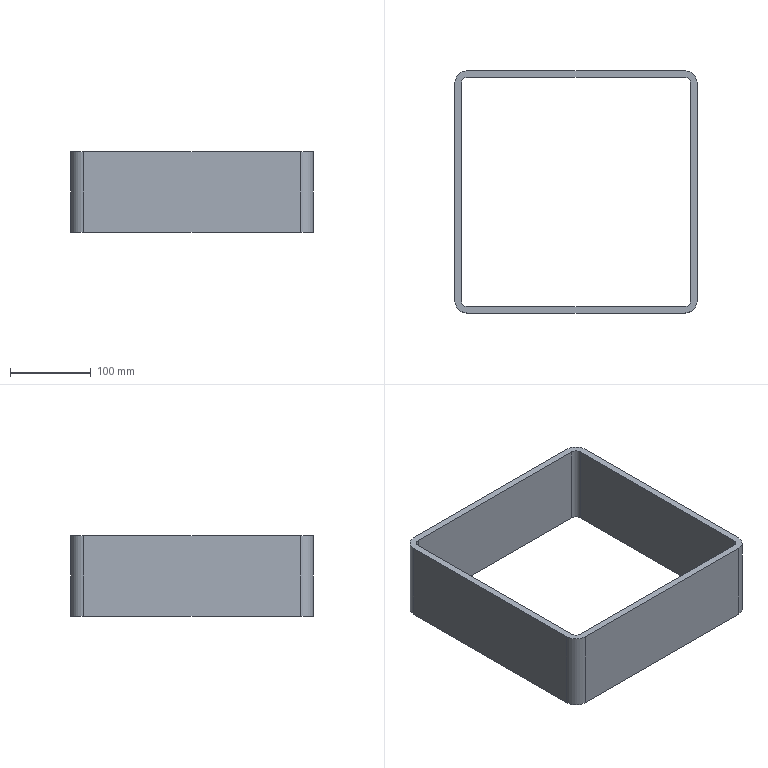Component | SolidWorks | TrolleyLeg-1_300 x 300 x 8-100-2 | 1 solid | 18 faces | box 300 x 300 x 100 mm | volume 917919 mm3 | plane 10 | cylinder 8 | commonest cylinder face diameters 32 x4 16 x4 | material Plain Carbon Steel
build123d program:
from build123d import *

# Parameters (mm, degrees)
BOSS_EXTRUDE1_DEPTH = 100


with BuildPart() as part:
    # Sketch1 → Boss-Extrude1 (new body)
    with BuildSketch(Plane.XY):
        with BuildLine():
            Line((-134, -150), (134, -150))
            ThreePointArc((134, -150), (145.314, -145.314), (150, -134))
            Line((150, -134), (150, 134))
            ThreePointArc((150, 134), (145.314, 145.314), (134, 150))
            Line((134, 150), (-134, 150))
            ThreePointArc((-134, 150), (-145.314, 145.314), (-150, 134))
            Line((-150, 134), (-150, -134))
            ThreePointArc((-150, -134), (-145.314, -145.314), (-134, -150))
        make_face()
        with BuildLine():
            Line((-134, -142), (134, -142))
            ThreePointArc((134, -142), (139.657, -139.657), (142, -134))
            Line((142, -134), (142, 134))
            ThreePointArc((142, 134), (139.657, 139.657), (134, 142))
            Line((134, 142), (-134, 142))
            ThreePointArc((-134, 142), (-139.657, 139.657), (-142, 134))
            Line((-142, 134), (-142, -134))
            ThreePointArc((-142, -134), (-139.657, -139.657), (-134, -142))
        make_face(mode=Mode.SUBTRACT)
    extrude(amount=BOSS_EXTRUDE1_DEPTH)


solid = part.part

# Placed as in the assembly
solid = solid.moved(Location((-2662.199, 1921.323, 3105.973), (0, 0, 0)))
STEP:
#1=COLOUR_RGB('',0.7922,0.8196,0.9333);
#2=FILL_AREA_STYLE_COLOUR('',#1);
#3=FILL_AREA_STYLE('',(#2));
#4=SURFACE_STYLE_FILL_AREA(#3);
#5=SURFACE_SIDE_STYLE('',(#4));
#6=SURFACE_STYLE_USAGE(.BOTH.,#5);
#7=PRESENTATION_STYLE_ASSIGNMENT((#6));
#8=CARTESIAN_POINT('',(-110.717,80.918,122.282));
#9=VERTEX_POINT('',#8);
#10=CARTESIAN_POINT('',(-110.087,81.548,122.282));
#11=VERTEX_POINT('',#10);
#12=CARTESIAN_POINT('',(-110.087,80.918,122.282));
#13=DIRECTION('',(0.,0.,-1.));
#14=DIRECTION('',(1.,0.,0.));
#15=AXIS2_PLACEMENT_3D('',#12,#13,#14);
#16=CIRCLE('',#15,0.6299);
#17=EDGE_CURVE('',#9,#11,#16,.T.);
#18=ORIENTED_EDGE('',*,*,#17,.T.);
#19=CARTESIAN_POINT('',(-99.535,81.548,122.282));
#20=VERTEX_POINT('',#19);
#21=CARTESIAN_POINT('',(-110.087,81.548,122.282));
#22=DIRECTION('',(1.,0.,0.));
#23=VECTOR('',#22,39.37);
#24=LINE('',#21,#23);
#25=EDGE_CURVE('',#11,#20,#24,.T.);
#26=ORIENTED_EDGE('',*,*,#25,.T.);
#27=CARTESIAN_POINT('',(-98.905,80.918,122.282));
#28=VERTEX_POINT('',#27);
#29=CARTESIAN_POINT('',(-99.535,80.918,122.282));
#30=DIRECTION('',(0.,0.,-1.));
#31=DIRECTION('',(1.,0.,0.));
#32=AXIS2_PLACEMENT_3D('',#29,#30,#31);
#33=CIRCLE('',#32,0.6299);
#34=EDGE_CURVE('',#20,#28,#33,.T.);
#35=ORIENTED_EDGE('',*,*,#34,.T.);
#36=CARTESIAN_POINT('',(-98.905,70.367,122.282));
#37=VERTEX_POINT('',#36);
#38=CARTESIAN_POINT('',(-98.905,70.367,122.282));
#39=DIRECTION('',(0.,1.,0.));
#40=VECTOR('',#39,39.37);
#41=LINE('',#38,#40);
#42=EDGE_CURVE('',#37,#28,#41,.T.);
#43=ORIENTED_EDGE('',*,*,#42,.F.);
#44=CARTESIAN_POINT('',(-99.535,69.737,122.282));
#45=VERTEX_POINT('',#44);
#46=CARTESIAN_POINT('',(-99.535,70.367,122.282));
#47=DIRECTION('',(0.,0.,-1.));
#48=DIRECTION('',(1.,0.,0.));
#49=AXIS2_PLACEMENT_3D('',#46,#47,#48);
#50=CIRCLE('',#49,0.6299);
#51=EDGE_CURVE('',#37,#45,#50,.T.);
#52=ORIENTED_EDGE('',*,*,#51,.T.);
#53=CARTESIAN_POINT('',(-110.087,69.737,122.282));
#54=VERTEX_POINT('',#53);
#55=CARTESIAN_POINT('',(-99.535,69.737,122.282));
#56=DIRECTION('',(-1.,0.,0.));
#57=VECTOR('',#56,39.37);
#58=LINE('',#55,#57);
#59=EDGE_CURVE('',#45,#54,#58,.T.);
#60=ORIENTED_EDGE('',*,*,#59,.T.);
#61=CARTESIAN_POINT('',(-110.717,70.367,122.282));
#62=VERTEX_POINT('',#61);
#63=CARTESIAN_POINT('',(-110.087,70.367,122.282));
#64=DIRECTION('',(0.,0.,-1.));
#65=DIRECTION('',(1.,0.,0.));
#66=AXIS2_PLACEMENT_3D('',#63,#64,#65);
#67=CIRCLE('',#66,0.6299);
#68=EDGE_CURVE('',#54,#62,#67,.T.);
#69=ORIENTED_EDGE('',*,*,#68,.T.);
#70=CARTESIAN_POINT('',(-110.717,80.918,122.282));
#71=DIRECTION('',(0.,-1.,0.));
#72=VECTOR('',#71,39.37);
#73=LINE('',#70,#72);
#74=EDGE_CURVE('',#9,#62,#73,.T.);
#75=ORIENTED_EDGE('',*,*,#74,.F.);
#76=EDGE_LOOP('',(#18,#26,#35,#43,#52,#60,#69,#75));
#77=FACE_OUTER_BOUND('',#76,.T.);
#78=CARTESIAN_POINT('',(-110.087,81.233,122.282));
#79=VERTEX_POINT('',#78);
#80=CARTESIAN_POINT('',(-99.535,81.233,122.282));
#81=VERTEX_POINT('',#80);
#82=CARTESIAN_POINT('',(-110.087,81.233,122.282));
#83=DIRECTION('',(1.,0.,0.));
#84=VECTOR('',#83,39.37);
#85=LINE('',#82,#84);
#86=EDGE_CURVE('',#79,#81,#85,.T.);
#87=ORIENTED_EDGE('',*,*,#86,.F.);
#88=CARTESIAN_POINT('',(-110.402,80.918,122.282));
#89=VERTEX_POINT('',#88);
#90=CARTESIAN_POINT('',(-110.087,80.918,122.282));
#91=DIRECTION('',(0.,0.,-1.));
#92=DIRECTION('',(1.,0.,0.));
#93=AXIS2_PLACEMENT_3D('',#90,#91,#92);
#94=CIRCLE('',#93,0.315);
#95=EDGE_CURVE('',#89,#79,#94,.T.);
#96=ORIENTED_EDGE('',*,*,#95,.F.);
#97=CARTESIAN_POINT('',(-110.402,70.367,122.282));
#98=VERTEX_POINT('',#97);
#99=CARTESIAN_POINT('',(-110.402,80.918,122.282));
#100=DIRECTION('',(0.,-1.,0.));
#101=VECTOR('',#100,39.37);
#102=LINE('',#99,#101);
#103=EDGE_CURVE('',#89,#98,#102,.T.);
#104=ORIENTED_EDGE('',*,*,#103,.T.);
#105=CARTESIAN_POINT('',(-110.087,70.052,122.282));
#106=VERTEX_POINT('',#105);
#107=CARTESIAN_POINT('',(-110.087,70.367,122.282));
#108=DIRECTION('',(0.,0.,-1.));
#109=DIRECTION('',(1.,0.,0.));
#110=AXIS2_PLACEMENT_3D('',#107,#108,#109);
#111=CIRCLE('',#110,0.315);
#112=EDGE_CURVE('',#106,#98,#111,.T.);
#113=ORIENTED_EDGE('',*,*,#112,.F.);
#114=CARTESIAN_POINT('',(-99.535,70.052,122.282));
#115=VERTEX_POINT('',#114);
#116=CARTESIAN_POINT('',(-99.535,70.052,122.282));
#117=DIRECTION('',(-1.,0.,0.));
#118=VECTOR('',#117,39.37);
#119=LINE('',#116,#118);
#120=EDGE_CURVE('',#115,#106,#119,.T.);
#121=ORIENTED_EDGE('',*,*,#120,.F.);
#122=CARTESIAN_POINT('',(-99.22,70.367,122.282));
#123=VERTEX_POINT('',#122);
#124=CARTESIAN_POINT('',(-99.535,70.367,122.282));
#125=DIRECTION('',(0.,0.,-1.));
#126=DIRECTION('',(1.,0.,0.));
#127=AXIS2_PLACEMENT_3D('',#124,#125,#126);
#128=CIRCLE('',#127,0.315);
#129=EDGE_CURVE('',#123,#115,#128,.T.);
#130=ORIENTED_EDGE('',*,*,#129,.F.);
#131=CARTESIAN_POINT('',(-99.22,80.918,122.282));
#132=VERTEX_POINT('',#131);
#133=CARTESIAN_POINT('',(-99.22,70.367,122.282));
#134=DIRECTION('',(0.,1.,0.));
#135=VECTOR('',#134,39.37);
#136=LINE('',#133,#135);
#137=EDGE_CURVE('',#123,#132,#136,.T.);
#138=ORIENTED_EDGE('',*,*,#137,.T.);
#139=CARTESIAN_POINT('',(-99.535,80.918,122.282));
#140=DIRECTION('',(0.,0.,-1.));
#141=DIRECTION('',(1.,0.,0.));
#142=AXIS2_PLACEMENT_3D('',#139,#140,#141);
#143=CIRCLE('',#142,0.315);
#144=EDGE_CURVE('',#81,#132,#143,.T.);
#145=ORIENTED_EDGE('',*,*,#144,.F.);
#146=EDGE_LOOP('',(#87,#96,#104,#113,#121,#130,#138,#145));
#147=FACE_BOUND('',#146,.T.);
#148=CARTESIAN_POINT('',(-110.087,80.918,122.282));
#149=DIRECTION('',(0.,0.,-1.));
#150=DIRECTION('',(1.,0.,0.));
#151=AXIS2_PLACEMENT_3D('',#148,#149,#150);
#152=PLANE('',#151);
#153=ADVANCED_FACE('',(#77,#147),#152,.T.);
#154=CARTESIAN_POINT('',(-110.717,80.918,126.219));
#155=VERTEX_POINT('',#154);
#156=CARTESIAN_POINT('',(-110.087,81.548,126.219));
#157=VERTEX_POINT('',#156);
#158=CARTESIAN_POINT('',(-110.087,80.918,126.219));
#159=DIRECTION('',(0.,0.,-1.));
#160=DIRECTION('',(1.,0.,0.));
#161=AXIS2_PLACEMENT_3D('',#158,#159,#160);
#162=CIRCLE('',#161,0.6299);
#163=EDGE_CURVE('',#155,#157,#162,.T.);
#164=ORIENTED_EDGE('',*,*,#163,.F.);
#165=CARTESIAN_POINT('',(-110.717,70.367,126.219));
#166=VERTEX_POINT('',#165);
#167=CARTESIAN_POINT('',(-110.717,80.918,126.219));
#168=DIRECTION('',(0.,-1.,0.));
#169=VECTOR('',#168,39.37);
#170=LINE('',#167,#169);
#171=EDGE_CURVE('',#155,#166,#170,.T.);
#172=ORIENTED_EDGE('',*,*,#171,.T.);
#173=CARTESIAN_POINT('',(-110.087,69.737,126.219));
#174=VERTEX_POINT('',#173);
#175=CARTESIAN_POINT('',(-110.087,70.367,126.219));
#176=DIRECTION('',(0.,0.,-1.));
#177=DIRECTION('',(1.,0.,0.));
#178=AXIS2_PLACEMENT_3D('',#175,#176,#177);
#179=CIRCLE('',#178,0.6299);
#180=EDGE_CURVE('',#174,#166,#179,.T.);
#181=ORIENTED_EDGE('',*,*,#180,.F.);
#182=CARTESIAN_POINT('',(-99.535,69.737,126.219));
#183=VERTEX_POINT('',#182);
#184=CARTESIAN_POINT('',(-99.535,69.737,126.219));
#185=DIRECTION('',(-1.,0.,0.));
#186=VECTOR('',#185,39.37);
#187=LINE('',#184,#186);
#188=EDGE_CURVE('',#183,#174,#187,.T.);
#189=ORIENTED_EDGE('',*,*,#188,.F.);
#190=CARTESIAN_POINT('',(-98.905,70.367,126.219));
#191=VERTEX_POINT('',#190);
#192=CARTESIAN_POINT('',(-99.535,70.367,126.219));
#193=DIRECTION('',(0.,0.,-1.));
#194=DIRECTION('',(1.,0.,0.));
#195=AXIS2_PLACEMENT_3D('',#192,#193,#194);
#196=CIRCLE('',#195,0.6299);
#197=EDGE_CURVE('',#191,#183,#196,.T.);
#198=ORIENTED_EDGE('',*,*,#197,.F.);
#199=CARTESIAN_POINT('',(-98.905,80.918,126.219));
#200=VERTEX_POINT('',#199);
#201=CARTESIAN_POINT('',(-98.905,70.367,126.219));
#202=DIRECTION('',(0.,1.,0.));
#203=VECTOR('',#202,39.37);
#204=LINE('',#201,#203);
#205=EDGE_CURVE('',#191,#200,#204,.T.);
#206=ORIENTED_EDGE('',*,*,#205,.T.);
#207=CARTESIAN_POINT('',(-99.535,81.548,126.219));
#208=VERTEX_POINT('',#207);
#209=CARTESIAN_POINT('',(-99.535,80.918,126.219));
#210=DIRECTION('',(0.,0.,-1.));
#211=DIRECTION('',(1.,0.,0.));
#212=AXIS2_PLACEMENT_3D('',#209,#210,#211);
#213=CIRCLE('',#212,0.6299);
#214=EDGE_CURVE('',#208,#200,#213,.T.);
#215=ORIENTED_EDGE('',*,*,#214,.F.);
#216=CARTESIAN_POINT('',(-110.087,81.548,126.219));
#217=DIRECTION('',(1.,0.,0.));
#218=VECTOR('',#217,39.37);
#219=LINE('',#216,#218);
#220=EDGE_CURVE('',#157,#208,#219,.T.);
#221=ORIENTED_EDGE('',*,*,#220,.F.);
#222=EDGE_LOOP('',(#164,#172,#181,#189,#198,#206,#215,#221));
#223=FACE_OUTER_BOUND('',#222,.T.);
#224=CARTESIAN_POINT('',(-110.402,80.918,126.219));
#225=VERTEX_POINT('',#224);
#226=CARTESIAN_POINT('',(-110.087,81.233,126.219));
#227=VERTEX_POINT('',#226);
#228=CARTESIAN_POINT('',(-110.087,80.918,126.219));
#229=DIRECTION('',(0.,0.,-1.));
#230=DIRECTION('',(1.,0.,0.));
#231=AXIS2_PLACEMENT_3D('',#228,#229,#230);
#232=CIRCLE('',#231,0.315);
#233=EDGE_CURVE('',#225,#227,#232,.T.);
#234=ORIENTED_EDGE('',*,*,#233,.T.);
#235=CARTESIAN_POINT('',(-99.535,81.233,126.219));
#236=VERTEX_POINT('',#235);
#237=CARTESIAN_POINT('',(-110.087,81.233,126.219));
#238=DIRECTION('',(1.,0.,0.));
#239=VECTOR('',#238,39.37);
#240=LINE('',#237,#239);
#241=EDGE_CURVE('',#227,#236,#240,.T.);
#242=ORIENTED_EDGE('',*,*,#241,.T.);
#243=CARTESIAN_POINT('',(-99.22,80.918,126.219));
#244=VERTEX_POINT('',#243);
#245=CARTESIAN_POINT('',(-99.535,80.918,126.219));
#246=DIRECTION('',(0.,0.,-1.));
#247=DIRECTION('',(1.,0.,0.));
#248=AXIS2_PLACEMENT_3D('',#245,#246,#247);
#249=CIRCLE('',#248,0.315);
#250=EDGE_CURVE('',#236,#244,#249,.T.);
#251=ORIENTED_EDGE('',*,*,#250,.T.);
#252=CARTESIAN_POINT('',(-99.22,70.367,126.219));
#253=VERTEX_POINT('',#252);
#254=CARTESIAN_POINT('',(-99.22,70.367,126.219));
#255=DIRECTION('',(0.,1.,0.));
#256=VECTOR('',#255,39.37);
#257=LINE('',#254,#256);
#258=EDGE_CURVE('',#253,#244,#257,.T.);
#259=ORIENTED_EDGE('',*,*,#258,.F.);
#260=CARTESIAN_POINT('',(-99.535,70.052,126.219));
#261=VERTEX_POINT('',#260);
#262=CARTESIAN_POINT('',(-99.535,70.367,126.219));
#263=DIRECTION('',(0.,0.,-1.));
#264=DIRECTION('',(1.,0.,0.));
#265=AXIS2_PLACEMENT_3D('',#262,#263,#264);
#266=CIRCLE('',#265,0.315);
#267=EDGE_CURVE('',#253,#261,#266,.T.);
#268=ORIENTED_EDGE('',*,*,#267,.T.);
#269=CARTESIAN_POINT('',(-110.087,70.052,126.219));
#270=VERTEX_POINT('',#269);
#271=CARTESIAN_POINT('',(-99.535,70.052,126.219));
#272=DIRECTION('',(-1.,0.,0.));
#273=VECTOR('',#272,39.37);
#274=LINE('',#271,#273);
#275=EDGE_CURVE('',#261,#270,#274,.T.);
#276=ORIENTED_EDGE('',*,*,#275,.T.);
#277=CARTESIAN_POINT('',(-110.402,70.367,126.219));
#278=VERTEX_POINT('',#277);
#279=CARTESIAN_POINT('',(-110.087,70.367,126.219));
#280=DIRECTION('',(0.,0.,-1.));
#281=DIRECTION('',(1.,0.,0.));
#282=AXIS2_PLACEMENT_3D('',#279,#280,#281);
#283=CIRCLE('',#282,0.315);
#284=EDGE_CURVE('',#270,#278,#283,.T.);
#285=ORIENTED_EDGE('',*,*,#284,.T.);
#286=CARTESIAN_POINT('',(-110.402,80.918,126.219));
#287=DIRECTION('',(0.,-1.,0.));
#288=VECTOR('',#287,39.37);
#289=LINE('',#286,#288);
#290=EDGE_CURVE('',#225,#278,#289,.T.);
#291=ORIENTED_EDGE('',*,*,#290,.F.);
#292=EDGE_LOOP('',(#234,#242,#251,#259,#268,#276,#285,#291));
#293=FACE_BOUND('',#292,.T.);
#294=CARTESIAN_POINT('',(-110.087,80.918,126.219));
#295=DIRECTION('',(0.,0.,-1.));
#296=DIRECTION('',(1.,0.,0.));
#297=AXIS2_PLACEMENT_3D('',#294,#295,#296);
#298=PLANE('',#297);
#299=ADVANCED_FACE('',(#223,#293),#298,.F.);
#300=ORIENTED_EDGE('',*,*,#163,.T.);
#301=CARTESIAN_POINT('',(-110.087,81.548,122.282));
#302=DIRECTION('',(0.,0.,1.));
#303=VECTOR('',#302,39.37);
#304=LINE('',#301,#303);
#305=EDGE_CURVE('',#11,#157,#304,.T.);
#306=ORIENTED_EDGE('',*,*,#305,.F.);
#307=ORIENTED_EDGE('',*,*,#17,.F.);
#308=CARTESIAN_POINT('',(-110.717,80.918,122.282));
#309=DIRECTION('',(0.,0.,1.));
#310=VECTOR('',#309,39.37);
#311=LINE('',#308,#310);
#312=EDGE_CURVE('',#9,#155,#311,.T.);
#313=ORIENTED_EDGE('',*,*,#312,.T.);
#314=EDGE_LOOP('',(#300,#306,#307,#313));
#315=FACE_OUTER_BOUND('',#314,.T.);
#316=CARTESIAN_POINT('',(-110.087,80.918,122.282));
#317=DIRECTION('',(0.,0.,1.));
#318=DIRECTION('',(-1.,0.,0.));
#319=AXIS2_PLACEMENT_3D('',#316,#317,#318);
#320=CYLINDRICAL_SURFACE('',#319,0.6299);
#321=ADVANCED_FACE('',(#315),#320,.T.);
#322=ORIENTED_EDGE('',*,*,#220,.T.);
#323=CARTESIAN_POINT('',(-99.535,81.548,122.282));
#324=DIRECTION('',(0.,0.,1.));
#325=VECTOR('',#324,39.37);
#326=LINE('',#323,#325);
#327=EDGE_CURVE('',#20,#208,#326,.T.);
#328=ORIENTED_EDGE('',*,*,#327,.F.);
#329=ORIENTED_EDGE('',*,*,#25,.F.);
#330=ORIENTED_EDGE('',*,*,#305,.T.);
#331=EDGE_LOOP('',(#322,#328,#329,#330));
#332=FACE_OUTER_BOUND('',#331,.T.);
#333=CARTESIAN_POINT('',(-110.087,81.548,122.282));
#334=DIRECTION('',(0.,-1.,0.));
#335=DIRECTION('',(0.,0.,-1.));
#336=AXIS2_PLACEMENT_3D('',#333,#334,#335);
#337=PLANE('',#336);
#338=ADVANCED_FACE('',(#332),#337,.F.);
#339=ORIENTED_EDGE('',*,*,#214,.T.);
#340=CARTESIAN_POINT('',(-98.905,80.918,122.282));
#341=DIRECTION('',(0.,0.,1.));
#342=VECTOR('',#341,39.37);
#343=LINE('',#340,#342);
#344=EDGE_CURVE('',#28,#200,#343,.T.);
#345=ORIENTED_EDGE('',*,*,#344,.F.);
#346=ORIENTED_EDGE('',*,*,#34,.F.);
#347=ORIENTED_EDGE('',*,*,#327,.T.);
#348=EDGE_LOOP('',(#339,#345,#346,#347));
#349=FACE_OUTER_BOUND('',#348,.T.);
#350=CARTESIAN_POINT('',(-99.535,80.918,122.282));
#351=DIRECTION('',(0.,0.,1.));
#352=DIRECTION('',(-1.,0.,0.));
#353=AXIS2_PLACEMENT_3D('',#350,#351,#352);
#354=CYLINDRICAL_SURFACE('',#353,0.6299);
#355=ADVANCED_FACE('',(#349),#354,.T.);
#356=ORIENTED_EDGE('',*,*,#205,.F.);
#357=CARTESIAN_POINT('',(-98.905,70.367,122.282));
#358=DIRECTION('',(0.,0.,1.));
#359=VECTOR('',#358,39.37);
#360=LINE('',#357,#359);
#361=EDGE_CURVE('',#37,#191,#360,.T.);
#362=ORIENTED_EDGE('',*,*,#361,.F.);
#363=ORIENTED_EDGE('',*,*,#42,.T.);
#364=ORIENTED_EDGE('',*,*,#344,.T.);
#365=EDGE_LOOP('',(#356,#362,#363,#364));
#366=FACE_OUTER_BOUND('',#365,.T.);
#367=CARTESIAN_POINT('',(-98.905,70.367,122.282));
#368=DIRECTION('',(1.,0.,0.));
#369=DIRECTION('',(0.,0.,1.));
#370=AXIS2_PLACEMENT_3D('',#367,#368,#369);
#371=PLANE('',#370);
#372=ADVANCED_FACE('',(#366),#371,.T.);
#373=ORIENTED_EDGE('',*,*,#197,.T.);
#374=CARTESIAN_POINT('',(-99.535,69.737,122.282));
#375=DIRECTION('',(0.,0.,1.));
#376=VECTOR('',#375,39.37);
#377=LINE('',#374,#376);
#378=EDGE_CURVE('',#45,#183,#377,.T.);
#379=ORIENTED_EDGE('',*,*,#378,.F.);
#380=ORIENTED_EDGE('',*,*,#51,.F.);
#381=ORIENTED_EDGE('',*,*,#361,.T.);
#382=EDGE_LOOP('',(#373,#379,#380,#381));
#383=FACE_OUTER_BOUND('',#382,.T.);
#384=CARTESIAN_POINT('',(-99.535,70.367,122.282));
#385=DIRECTION('',(0.,0.,1.));
#386=DIRECTION('',(-1.,0.,0.));
#387=AXIS2_PLACEMENT_3D('',#384,#385,#386);
#388=CYLINDRICAL_SURFACE('',#387,0.6299);
#389=ADVANCED_FACE('',(#383),#388,.T.);
#390=ORIENTED_EDGE('',*,*,#188,.T.);
#391=CARTESIAN_POINT('',(-110.087,69.737,122.282));
#392=DIRECTION('',(0.,0.,1.));
#393=VECTOR('',#392,39.37);
#394=LINE('',#391,#393);
#395=EDGE_CURVE('',#54,#174,#394,.T.);
#396=ORIENTED_EDGE('',*,*,#395,.F.);
#397=ORIENTED_EDGE('',*,*,#59,.F.);
#398=ORIENTED_EDGE('',*,*,#378,.T.);
#399=EDGE_LOOP('',(#390,#396,#397,#398));
#400=FACE_OUTER_BOUND('',#399,.T.);
#401=CARTESIAN_POINT('',(-99.535,69.737,122.282));
#402=DIRECTION('',(0.,1.,0.));
#403=DIRECTION('',(0.,0.,1.));
#404=AXIS2_PLACEMENT_3D('',#401,#402,#403);
#405=PLANE('',#404);
#406=ADVANCED_FACE('',(#400),#405,.F.);
#407=ORIENTED_EDGE('',*,*,#180,.T.);
#408=CARTESIAN_POINT('',(-110.717,70.367,122.282));
#409=DIRECTION('',(0.,0.,1.));
#410=VECTOR('',#409,39.37);
#411=LINE('',#408,#410);
#412=EDGE_CURVE('',#62,#166,#411,.T.);
#413=ORIENTED_EDGE('',*,*,#412,.F.);
#414=ORIENTED_EDGE('',*,*,#68,.F.);
#415=ORIENTED_EDGE('',*,*,#395,.T.);
#416=EDGE_LOOP('',(#407,#413,#414,#415));
#417=FACE_OUTER_BOUND('',#416,.T.);
#418=CARTESIAN_POINT('',(-110.087,70.367,122.282));
#419=DIRECTION('',(0.,0.,1.));
#420=DIRECTION('',(-1.,0.,0.));
#421=AXIS2_PLACEMENT_3D('',#418,#419,#420);
#422=CYLINDRICAL_SURFACE('',#421,0.6299);
#423=ADVANCED_FACE('',(#417),#422,.T.);
#424=ORIENTED_EDGE('',*,*,#171,.F.);
#425=ORIENTED_EDGE('',*,*,#312,.F.);
#426=ORIENTED_EDGE('',*,*,#74,.T.);
#427=ORIENTED_EDGE('',*,*,#412,.T.);
#428=EDGE_LOOP('',(#424,#425,#426,#427));
#429=FACE_OUTER_BOUND('',#428,.T.);
#430=CARTESIAN_POINT('',(-110.717,80.918,122.282));
#431=DIRECTION('',(-1.,0.,0.));
#432=DIRECTION('',(0.,0.,-1.));
#433=AXIS2_PLACEMENT_3D('',#430,#431,#432);
#434=PLANE('',#433);
#435=ADVANCED_FACE('',(#429),#434,.T.);
#436=ORIENTED_EDGE('',*,*,#233,.F.);
#437=CARTESIAN_POINT('',(-110.402,80.918,122.282));
#438=DIRECTION('',(0.,0.,1.));
#439=VECTOR('',#438,39.37);
#440=LINE('',#437,#439);
#441=EDGE_CURVE('',#89,#225,#440,.T.);
#442=ORIENTED_EDGE('',*,*,#441,.F.);
#443=ORIENTED_EDGE('',*,*,#95,.T.);
#444=CARTESIAN_POINT('',(-110.087,81.233,122.282));
#445=DIRECTION('',(0.,0.,1.));
#446=VECTOR('',#445,39.37);
#447=LINE('',#444,#446);
#448=EDGE_CURVE('',#79,#227,#447,.T.);
#449=ORIENTED_EDGE('',*,*,#448,.T.);
#450=EDGE_LOOP('',(#436,#442,#443,#449));
#451=FACE_OUTER_BOUND('',#450,.T.);
#452=CARTESIAN_POINT('',(-110.087,80.918,122.282));
#453=DIRECTION('',(0.,0.,1.));
#454=DIRECTION('',(-1.,0.,0.));
#455=AXIS2_PLACEMENT_3D('',#452,#453,#454);
#456=CYLINDRICAL_SURFACE('',#455,0.315);
#457=ADVANCED_FACE('',(#451),#456,.F.);
#458=ORIENTED_EDGE('',*,*,#241,.F.);
#459=ORIENTED_EDGE('',*,*,#448,.F.);
#460=ORIENTED_EDGE('',*,*,#86,.T.);
#461=CARTESIAN_POINT('',(-99.535,81.233,122.282));
#462=DIRECTION('',(0.,0.,1.));
#463=VECTOR('',#462,39.37);
#464=LINE('',#461,#463);
#465=EDGE_CURVE('',#81,#236,#464,.T.);
#466=ORIENTED_EDGE('',*,*,#465,.T.);
#467=EDGE_LOOP('',(#458,#459,#460,#466));
#468=FACE_OUTER_BOUND('',#467,.T.);
#469=CARTESIAN_POINT('',(-110.087,81.233,122.282));
#470=DIRECTION('',(0.,-1.,0.));
#471=DIRECTION('',(0.,0.,-1.));
#472=AXIS2_PLACEMENT_3D('',#469,#470,#471);
#473=PLANE('',#472);
#474=ADVANCED_FACE('',(#468),#473,.T.);
#475=ORIENTED_EDGE('',*,*,#250,.F.);
#476=ORIENTED_EDGE('',*,*,#465,.F.);
#477=ORIENTED_EDGE('',*,*,#144,.T.);
#478=CARTESIAN_POINT('',(-99.22,80.918,122.282));
#479=DIRECTION('',(0.,0.,1.));
#480=VECTOR('',#479,39.37);
#481=LINE('',#478,#480);
#482=EDGE_CURVE('',#132,#244,#481,.T.);
#483=ORIENTED_EDGE('',*,*,#482,.T.);
#484=EDGE_LOOP('',(#475,#476,#477,#483));
#485=FACE_OUTER_BOUND('',#484,.T.);
#486=CARTESIAN_POINT('',(-99.535,80.918,122.282));
#487=DIRECTION('',(0.,0.,1.));
#488=DIRECTION('',(-1.,0.,0.));
#489=AXIS2_PLACEMENT_3D('',#486,#487,#488);
#490=CYLINDRICAL_SURFACE('',#489,0.315);
#491=ADVANCED_FACE('',(#485),#490,.F.);
#492=ORIENTED_EDGE('',*,*,#258,.T.);
#493=ORIENTED_EDGE('',*,*,#482,.F.);
#494=ORIENTED_EDGE('',*,*,#137,.F.);
#495=CARTESIAN_POINT('',(-99.22,70.367,122.282));
#496=DIRECTION('',(0.,0.,1.));
#497=VECTOR('',#496,39.37);
#498=LINE('',#495,#497);
#499=EDGE_CURVE('',#123,#253,#498,.T.);
#500=ORIENTED_EDGE('',*,*,#499,.T.);
#501=EDGE_LOOP('',(#492,#493,#494,#500));
#502=FACE_OUTER_BOUND('',#501,.T.);
#503=CARTESIAN_POINT('',(-99.22,70.367,122.282));
#504=DIRECTION('',(1.,0.,0.));
#505=DIRECTION('',(0.,0.,1.));
#506=AXIS2_PLACEMENT_3D('',#503,#504,#505);
#507=PLANE('',#506);
#508=ADVANCED_FACE('',(#502),#507,.F.);
#509=ORIENTED_EDGE('',*,*,#267,.F.);
#510=ORIENTED_EDGE('',*,*,#499,.F.);
#511=ORIENTED_EDGE('',*,*,#129,.T.);
#512=CARTESIAN_POINT('',(-99.535,70.052,122.282));
#513=DIRECTION('',(0.,0.,1.));
#514=VECTOR('',#513,39.37);
#515=LINE('',#512,#514);
#516=EDGE_CURVE('',#115,#261,#515,.T.);
#517=ORIENTED_EDGE('',*,*,#516,.T.);
#518=EDGE_LOOP('',(#509,#510,#511,#517));
#519=FACE_OUTER_BOUND('',#518,.T.);
#520=CARTESIAN_POINT('',(-99.535,70.367,122.282));
#521=DIRECTION('',(0.,0.,1.));
#522=DIRECTION('',(-1.,0.,0.));
#523=AXIS2_PLACEMENT_3D('',#520,#521,#522);
#524=CYLINDRICAL_SURFACE('',#523,0.315);
#525=ADVANCED_FACE('',(#519),#524,.F.);
#526=ORIENTED_EDGE('',*,*,#275,.F.);
#527=ORIENTED_EDGE('',*,*,#516,.F.);
#528=ORIENTED_EDGE('',*,*,#120,.T.);
#529=CARTESIAN_POINT('',(-110.087,70.052,122.282));
#530=DIRECTION('',(0.,0.,1.));
#531=VECTOR('',#530,39.37);
#532=LINE('',#529,#531);
#533=EDGE_CURVE('',#106,#270,#532,.T.);
#534=ORIENTED_EDGE('',*,*,#533,.T.);
#535=EDGE_LOOP('',(#526,#527,#528,#534));
#536=FACE_OUTER_BOUND('',#535,.T.);
#537=CARTESIAN_POINT('',(-99.535,70.052,122.282));
#538=DIRECTION('',(0.,1.,0.));
#539=DIRECTION('',(0.,0.,1.));
#540=AXIS2_PLACEMENT_3D('',#537,#538,#539);
#541=PLANE('',#540);
#542=ADVANCED_FACE('',(#536),#541,.T.);
#543=ORIENTED_EDGE('',*,*,#284,.F.);
#544=ORIENTED_EDGE('',*,*,#533,.F.);
#545=ORIENTED_EDGE('',*,*,#112,.T.);
#546=CARTESIAN_POINT('',(-110.402,70.367,122.282));
#547=DIRECTION('',(0.,0.,1.));
#548=VECTOR('',#547,39.37);
#549=LINE('',#546,#548);
#550=EDGE_CURVE('',#98,#278,#549,.T.);
#551=ORIENTED_EDGE('',*,*,#550,.T.);
#552=EDGE_LOOP('',(#543,#544,#545,#551));
#553=FACE_OUTER_BOUND('',#552,.T.);
#554=CARTESIAN_POINT('',(-110.087,70.367,122.282));
#555=DIRECTION('',(0.,0.,1.));
#556=DIRECTION('',(-1.,0.,0.));
#557=AXIS2_PLACEMENT_3D('',#554,#555,#556);
#558=CYLINDRICAL_SURFACE('',#557,0.315);
#559=ADVANCED_FACE('',(#553),#558,.F.);
#560=ORIENTED_EDGE('',*,*,#290,.T.);
#561=ORIENTED_EDGE('',*,*,#550,.F.);
#562=ORIENTED_EDGE('',*,*,#103,.F.);
#563=ORIENTED_EDGE('',*,*,#441,.T.);
#564=EDGE_LOOP('',(#560,#561,#562,#563));
#565=FACE_OUTER_BOUND('',#564,.T.);
#566=CARTESIAN_POINT('',(-110.402,80.918,122.282));
#567=DIRECTION('',(-1.,0.,0.));
#568=DIRECTION('',(0.,0.,-1.));
#569=AXIS2_PLACEMENT_3D('',#566,#567,#568);
#570=PLANE('',#569);
#571=ADVANCED_FACE('',(#565),#570,.F.);
#572=CLOSED_SHELL('',(#153,#299,#321,#338,#355,#372,#389,#406,#423,#435,#457,#474,#491,#508,#525,#542,#559,#571));
#573=MANIFOLD_SOLID_BREP('',#572);
#574=STYLED_ITEM('',(#7),#573);
#575=(LENGTH_UNIT()NAMED_UNIT(*)SI_UNIT($,.METRE.));
#576=LENGTH_MEASURE_WITH_UNIT(LENGTH_MEASURE(0.0254),#575);
#577=DIMENSIONAL_EXPONENTS(1.,0.,0.,0.,0.,0.,0.);
#578=(CONVERSION_BASED_UNIT('',#576)LENGTH_UNIT()NAMED_UNIT(#577));
#579=UNCERTAINTY_MEASURE_WITH_UNIT(LENGTH_MEASURE(0.00001),#578,'','');
#580=(NAMED_UNIT(*)PLANE_ANGLE_UNIT()SI_UNIT($,.RADIAN.));
#581=(NAMED_UNIT(*)SI_UNIT($,.STERADIAN.)SOLID_ANGLE_UNIT());
#582=(GEOMETRIC_REPRESENTATION_CONTEXT(3)GLOBAL_UNCERTAINTY_ASSIGNED_CONTEXT((#579))GLOBAL_UNIT_ASSIGNED_CONTEXT((#578,#580,#581))REPRESENTATION_CONTEXT('',''));
#583=MECHANICAL_DESIGN_GEOMETRIC_PRESENTATION_REPRESENTATION('',(#574),#582);
#584=PRESENTATION_LAYER_ASSIGNMENT('','',(#574));
#585=CARTESIAN_POINT('',(0.,0.,0.));
#586=DIRECTION('',(0.,0.,1.));
#587=DIRECTION('',(1.,0.,0.));
#588=AXIS2_PLACEMENT_3D('',#585,#586,#587);
#589=(LENGTH_UNIT()NAMED_UNIT(*)SI_UNIT($,.METRE.));
#590=LENGTH_MEASURE_WITH_UNIT(LENGTH_MEASURE(0.0254),#589);
#591=DIMENSIONAL_EXPONENTS(1.,0.,0.,0.,0.,0.,0.);
#592=(CONVERSION_BASED_UNIT('',#590)LENGTH_UNIT()NAMED_UNIT(#591));
#593=UNCERTAINTY_MEASURE_WITH_UNIT(LENGTH_MEASURE(0.00001),#592,'','');
#594=(NAMED_UNIT(*)PLANE_ANGLE_UNIT()SI_UNIT($,.RADIAN.));
#595=(NAMED_UNIT(*)SI_UNIT($,.STERADIAN.)SOLID_ANGLE_UNIT());
#596=(GEOMETRIC_REPRESENTATION_CONTEXT(3)GLOBAL_UNCERTAINTY_ASSIGNED_CONTEXT((#593))GLOBAL_UNIT_ASSIGNED_CONTEXT((#592,#594,#595))REPRESENTATION_CONTEXT('',''));
#597=ADVANCED_BREP_SHAPE_REPRESENTATION('',(#573,#588),#596);